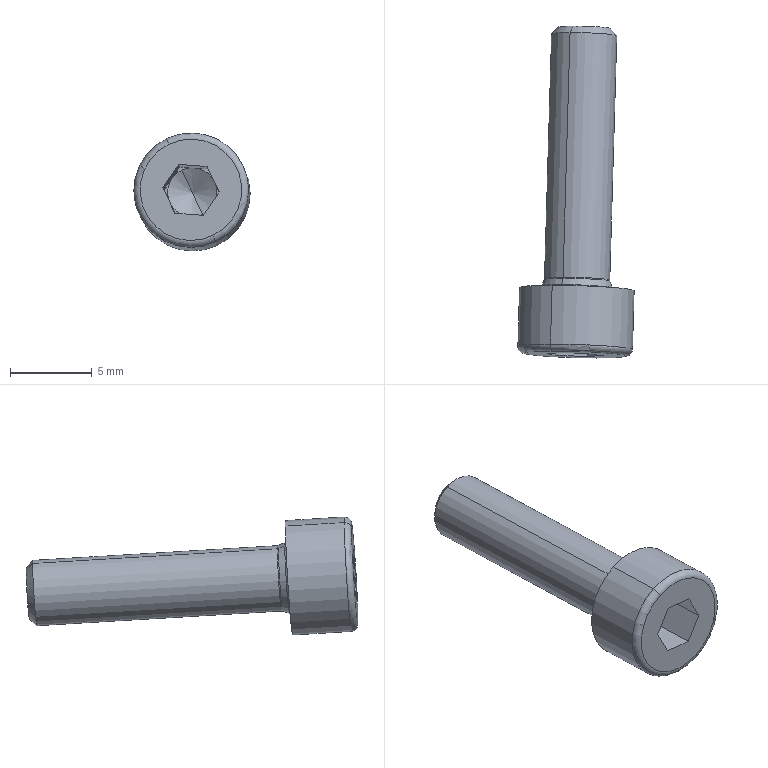Component | SolidWorks | HTCPA32_S5M100_12-1_Slotted_head_cap_screw_ISO_4762_M4x16-1 | 1 solid | 31 faces | box 7.1 x 20.27 x 7.2 mm | volume 332 mm3 | plane 15 | cone 6 | torus 6 | cylinder 4 | commonest cylinder face diameters 4 x2 7 x2
STEP:
#1=COLOUR_RGB('',0.7922,0.8196,0.9333);
#2=FILL_AREA_STYLE_COLOUR('',#1);
#3=FILL_AREA_STYLE('',(#2));
#4=SURFACE_STYLE_FILL_AREA(#3);
#5=SURFACE_SIDE_STYLE('',(#4));
#6=SURFACE_STYLE_USAGE(.BOTH.,#5);
#7=PRESENTATION_STYLE_ASSIGNMENT((#6));
#8=CARTESIAN_POINT('',(-1.2,11.445,21.934));
#9=VERTEX_POINT('',#8);
#10=CARTESIAN_POINT('',(-1.226,11.415,21.989));
#11=VERTEX_POINT('',#10);
#12=CARTESIAN_POINT('',(-1.226,11.415,21.989));
#13=DIRECTION('',(-0.3875,-0.4412,0.8094));
#14=VECTOR('',#13,39.37);
#15=LINE('',#12,#14);
#16=EDGE_CURVE('',#9,#11,#15,.T.);
#17=ORIENTED_EDGE('',*,*,#16,.F.);
#18=CARTESIAN_POINT('',(-1.175,11.407,21.883));
#19=VERTEX_POINT('',#18);
#20=CARTESIAN_POINT('',(-1.175,11.407,21.883));
#21=DIRECTION('',(0.3587,-0.5566,-0.7494));
#22=VECTOR('',#21,39.37);
#23=LINE('',#20,#22);
#24=EDGE_CURVE('',#9,#19,#23,.T.);
#25=ORIENTED_EDGE('',*,*,#24,.T.);
#26=CARTESIAN_POINT('',(-1.152,11.408,21.903));
#27=VERTEX_POINT('',#26);
#28=CARTESIAN_POINT('',(-1.201,11.411,21.936));
#29=DIRECTION('',(-0.02875,-0.9978,0.06006));
#30=DIRECTION('',(-0.4308,0.06659,0.9));
#31=AXIS2_PLACEMENT_3D('',#28,#29,#30);
#32=CIRCLE('',#31,0.05906);
#33=EDGE_CURVE('',#19,#27,#32,.T.);
#34=ORIENTED_EDGE('',*,*,#33,.T.);
#35=CARTESIAN_POINT('',(-1.147,11.411,21.962));
#36=VERTEX_POINT('',#35);
#37=CARTESIAN_POINT('',(-1.201,11.411,21.936));
#38=DIRECTION('',(-0.02875,-0.9978,0.06006));
#39=DIRECTION('',(-0.4308,0.06659,0.9));
#40=AXIS2_PLACEMENT_3D('',#37,#38,#39);
#41=CIRCLE('',#40,0.05906);
#42=EDGE_CURVE('',#27,#36,#41,.T.);
#43=ORIENTED_EDGE('',*,*,#42,.T.);
#44=CARTESIAN_POINT('',(-1.196,11.415,21.995));
#45=VERTEX_POINT('',#44);
#46=CARTESIAN_POINT('',(-1.201,11.411,21.936));
#47=DIRECTION('',(-0.02875,-0.9978,0.06006));
#48=DIRECTION('',(-0.4308,0.06659,0.9));
#49=AXIS2_PLACEMENT_3D('',#46,#47,#48);
#50=CIRCLE('',#49,0.05906);
#51=EDGE_CURVE('',#36,#45,#50,.T.);
#52=ORIENTED_EDGE('',*,*,#51,.T.);
#53=CARTESIAN_POINT('',(-1.201,11.411,21.936));
#54=DIRECTION('',(-0.02875,-0.9978,0.06006));
#55=DIRECTION('',(-0.4308,0.06659,0.9));
#56=AXIS2_PLACEMENT_3D('',#53,#54,#55);
#57=CIRCLE('',#56,0.05906);
#58=EDGE_CURVE('',#45,#11,#57,.T.);
#59=ORIENTED_EDGE('',*,*,#58,.T.);
#60=EDGE_LOOP('',(#17,#25,#34,#43,#52,#59));
#61=FACE_OUTER_BOUND('',#60,.T.);
#62=CARTESIAN_POINT('',(-1.201,11.411,21.936));
#63=DIRECTION('',(-0.02875,-0.9978,0.06006));
#64=DIRECTION('',(-0.4308,0.06659,0.9));
#65=AXIS2_PLACEMENT_3D('',#62,#63,#64);
#66=CONICAL_SURFACE('',#65,0.05906,1.047);
#67=ADVANCED_FACE('',(#61),#66,.F.);
#68=CARTESIAN_POINT('',(-1.208,12.099,21.951));
#69=VERTEX_POINT('',#68);
#70=CARTESIAN_POINT('',(-1.154,12.091,21.839));
#71=VERTEX_POINT('',#70);
#72=CARTESIAN_POINT('',(-1.181,12.095,21.895));
#73=DIRECTION('',(-0.02875,-0.9978,0.06006));
#74=DIRECTION('',(-0.4308,0.06659,0.9));
#75=AXIS2_PLACEMENT_3D('',#72,#73,#74);
#76=CIRCLE('',#75,0.06183);
#77=EDGE_CURVE('',#69,#71,#76,.T.);
#78=ORIENTED_EDGE('',*,*,#77,.T.);
#79=CARTESIAN_POINT('',(-1.147,12.073,21.825));
#80=VERTEX_POINT('',#79);
#81=CARTESIAN_POINT('',(-1.154,12.091,21.839));
#82=DIRECTION('',(0.2843,-0.7526,-0.5939));
#83=VECTOR('',#82,39.37);
#84=LINE('',#81,#83);
#85=EDGE_CURVE('',#71,#80,#84,.T.);
#86=ORIENTED_EDGE('',*,*,#85,.T.);
#87=CARTESIAN_POINT('',(-1.215,12.083,21.967));
#88=VERTEX_POINT('',#87);
#89=CARTESIAN_POINT('',(-1.181,12.078,21.896));
#90=DIRECTION('',(-0.02875,-0.9978,0.06006));
#91=DIRECTION('',(-0.4308,0.06659,0.9));
#92=AXIS2_PLACEMENT_3D('',#89,#90,#91);
#93=CIRCLE('',#92,0.07874);
#94=EDGE_CURVE('',#88,#80,#93,.T.);
#95=ORIENTED_EDGE('',*,*,#94,.F.);
#96=CARTESIAN_POINT('',(-1.208,12.099,21.951));
#97=DIRECTION('',(-0.325,-0.6585,0.6788));
#98=VECTOR('',#97,39.37);
#99=LINE('',#96,#98);
#100=EDGE_CURVE('',#69,#88,#99,.T.);
#101=ORIENTED_EDGE('',*,*,#100,.F.);
#102=EDGE_LOOP('',(#78,#86,#95,#101));
#103=FACE_OUTER_BOUND('',#102,.T.);
#104=CARTESIAN_POINT('',(-1.181,12.095,21.895));
#105=DIRECTION('',(-0.02875,-0.9978,0.06006));
#106=DIRECTION('',(-0.4308,0.06659,0.9));
#107=AXIS2_PLACEMENT_3D('',#104,#105,#106);
#108=CONICAL_SURFACE('',#107,0.06183,0.7854);
#109=ADVANCED_FACE('',(#103),#108,.T.);
#110=ORIENTED_EDGE('',*,*,#94,.T.);
#111=CARTESIAN_POINT('',(-1.164,11.485,21.861));
#112=VERTEX_POINT('',#111);
#113=CARTESIAN_POINT('',(-1.147,12.09,21.824));
#114=DIRECTION('',(-0.02875,-0.9978,0.06006));
#115=VECTOR('',#114,39.37);
#116=LINE('',#113,#115);
#117=EDGE_CURVE('',#80,#112,#116,.T.);
#118=ORIENTED_EDGE('',*,*,#117,.T.);
#119=CARTESIAN_POINT('',(-1.232,11.495,22.002));
#120=VERTEX_POINT('',#119);
#121=CARTESIAN_POINT('',(-1.198,11.49,21.931));
#122=DIRECTION('',(-0.02875,-0.9978,0.06006));
#123=DIRECTION('',(-0.4308,0.06659,0.9));
#124=AXIS2_PLACEMENT_3D('',#121,#122,#123);
#125=CIRCLE('',#124,0.07874);
#126=EDGE_CURVE('',#120,#112,#125,.T.);
#127=ORIENTED_EDGE('',*,*,#126,.F.);
#128=CARTESIAN_POINT('',(-1.215,12.1,21.966));
#129=DIRECTION('',(-0.02875,-0.9978,0.06006));
#130=VECTOR('',#129,39.37);
#131=LINE('',#128,#130);
#132=EDGE_CURVE('',#88,#120,#131,.T.);
#133=ORIENTED_EDGE('',*,*,#132,.F.);
#134=EDGE_LOOP('',(#110,#118,#127,#133));
#135=FACE_OUTER_BOUND('',#134,.T.);
#136=CARTESIAN_POINT('',(-1.181,12.095,21.895));
#137=DIRECTION('',(-0.02875,-0.9978,0.06006));
#138=DIRECTION('',(-0.4308,0.06659,0.9));
#139=AXIS2_PLACEMENT_3D('',#136,#137,#138);
#140=CYLINDRICAL_SURFACE('',#139,0.07874);
#141=ADVANCED_FACE('',(#135),#140,.T.);
#142=CARTESIAN_POINT('',(-1.164,11.482,21.86));
#143=VERTEX_POINT('',#142);
#144=CARTESIAN_POINT('',(-1.233,11.492,22.003));
#145=VERTEX_POINT('',#144);
#146=CARTESIAN_POINT('',(-1.198,11.487,21.932));
#147=DIRECTION('',(-0.02875,-0.9978,0.06006));
#148=DIRECTION('',(-0.4308,0.06659,0.9));
#149=AXIS2_PLACEMENT_3D('',#146,#147,#148);
#150=CIRCLE('',#149,0.07924);
#151=EDGE_CURVE('',#143,#145,#150,.T.);
#152=ORIENTED_EDGE('',*,*,#151,.F.);
#153=CARTESIAN_POINT('',(-1.161,11.484,21.853));
#154=DIRECTION('',(-0.902,0.,-0.4318));
#155=DIRECTION('',(-0.4318,0.,0.902));
#156=AXIS2_PLACEMENT_3D('',#153,#154,#155);
#157=CIRCLE('',#156,0.007874);
#158=EDGE_CURVE('',#143,#112,#157,.T.);
#159=ORIENTED_EDGE('',*,*,#158,.T.);
#160=CARTESIAN_POINT('',(-1.198,11.49,21.931));
#161=DIRECTION('',(-0.02875,-0.9978,0.06006));
#162=DIRECTION('',(-0.4308,0.06659,0.9));
#163=AXIS2_PLACEMENT_3D('',#160,#161,#162);
#164=CIRCLE('',#163,0.07874);
#165=EDGE_CURVE('',#112,#120,#164,.T.);
#166=ORIENTED_EDGE('',*,*,#165,.T.);
#167=CARTESIAN_POINT('',(-1.236,11.496,22.009));
#168=DIRECTION('',(0.902,-0.,0.4318));
#169=DIRECTION('',(0.4318,0.,-0.902));
#170=AXIS2_PLACEMENT_3D('',#167,#168,#169);
#171=CIRCLE('',#170,0.007874);
#172=EDGE_CURVE('',#145,#120,#171,.T.);
#173=ORIENTED_EDGE('',*,*,#172,.F.);
#174=EDGE_LOOP('',(#152,#159,#166,#173));
#175=FACE_OUTER_BOUND('',#174,.T.);
#176=CARTESIAN_POINT('',(-1.198,11.49,21.931));
#177=DIRECTION('',(-0.02875,-0.9978,0.06006));
#178=DIRECTION('',(-0.4308,0.06659,0.9));
#179=AXIS2_PLACEMENT_3D('',#176,#177,#178);
#180=TOROIDAL_SURFACE('',#179,0.08661,0.007874);
#181=ADVANCED_FACE('',(#175),#180,.F.);
#182=CARTESIAN_POINT('',(-1.198,11.487,21.932));
#183=DIRECTION('',(-0.02875,-0.9978,0.06006));
#184=DIRECTION('',(-0.4308,0.06659,0.9));
#185=AXIS2_PLACEMENT_3D('',#182,#183,#184);
#186=CIRCLE('',#185,0.07924);
#187=EDGE_CURVE('',#145,#143,#186,.T.);
#188=ORIENTED_EDGE('',*,*,#187,.T.);
#189=CARTESIAN_POINT('',(-1.162,11.466,21.856));
#190=VERTEX_POINT('',#189);
#191=CARTESIAN_POINT('',(-1.164,11.482,21.86));
#192=DIRECTION('',(0.1244,-0.9576,-0.2598));
#193=VECTOR('',#192,39.37);
#194=LINE('',#191,#193);
#195=EDGE_CURVE('',#143,#190,#194,.T.);
#196=ORIENTED_EDGE('',*,*,#195,.T.);
#197=CARTESIAN_POINT('',(-1.236,11.477,22.009));
#198=VERTEX_POINT('',#197);
#199=CARTESIAN_POINT('',(-1.199,11.471,21.933));
#200=DIRECTION('',(-0.02875,-0.9978,0.06006));
#201=DIRECTION('',(-0.4308,0.06659,0.9));
#202=AXIS2_PLACEMENT_3D('',#199,#200,#201);
#203=CIRCLE('',#202,0.08515);
#204=EDGE_CURVE('',#198,#190,#203,.T.);
#205=ORIENTED_EDGE('',*,*,#204,.F.);
#206=CARTESIAN_POINT('',(-1.233,11.492,22.003));
#207=DIRECTION('',(-0.1782,-0.9109,0.3722));
#208=VECTOR('',#207,39.37);
#209=LINE('',#206,#208);
#210=EDGE_CURVE('',#145,#198,#209,.T.);
#211=ORIENTED_EDGE('',*,*,#210,.F.);
#212=EDGE_LOOP('',(#188,#196,#205,#211));
#213=FACE_OUTER_BOUND('',#212,.T.);
#214=CARTESIAN_POINT('',(-1.198,11.487,21.932));
#215=DIRECTION('',(-0.02875,-0.9978,0.06006));
#216=DIRECTION('',(-0.4308,0.06659,0.9));
#217=AXIS2_PLACEMENT_3D('',#214,#215,#216);
#218=CONICAL_SURFACE('',#217,0.07924,0.3588);
#219=ADVANCED_FACE('',(#213),#218,.T.);
#220=CARTESIAN_POINT('',(-1.159,11.46,21.85));
#221=VERTEX_POINT('',#220);
#222=CARTESIAN_POINT('',(-1.239,11.472,22.016));
#223=VERTEX_POINT('',#222);
#224=CARTESIAN_POINT('',(-1.199,11.466,21.933));
#225=DIRECTION('',(-0.02875,-0.9978,0.06006));
#226=DIRECTION('',(-0.4308,0.06659,0.9));
#227=AXIS2_PLACEMENT_3D('',#224,#225,#226);
#228=CIRCLE('',#227,0.09252);
#229=EDGE_CURVE('',#221,#223,#228,.T.);
#230=ORIENTED_EDGE('',*,*,#229,.F.);
#231=CARTESIAN_POINT('',(-1.159,11.468,21.849));
#232=DIRECTION('',(-0.902,0.,-0.4318));
#233=DIRECTION('',(-0.4318,0.,0.902));
#234=AXIS2_PLACEMENT_3D('',#231,#232,#233);
#235=CIRCLE('',#234,0.007874);
#236=EDGE_CURVE('',#221,#190,#235,.T.);
#237=ORIENTED_EDGE('',*,*,#236,.T.);
#238=CARTESIAN_POINT('',(-1.199,11.471,21.933));
#239=DIRECTION('',(-0.02875,-0.9978,0.06006));
#240=DIRECTION('',(-0.4308,0.06659,0.9));
#241=AXIS2_PLACEMENT_3D('',#238,#239,#240);
#242=CIRCLE('',#241,0.08515);
#243=EDGE_CURVE('',#190,#198,#242,.T.);
#244=ORIENTED_EDGE('',*,*,#243,.T.);
#245=CARTESIAN_POINT('',(-1.239,11.48,22.016));
#246=DIRECTION('',(0.902,-0.,0.4318));
#247=DIRECTION('',(0.4318,0.,-0.902));
#248=AXIS2_PLACEMENT_3D('',#245,#246,#247);
#249=CIRCLE('',#248,0.007874);
#250=EDGE_CURVE('',#223,#198,#249,.T.);
#251=ORIENTED_EDGE('',*,*,#250,.F.);
#252=EDGE_LOOP('',(#230,#237,#244,#251));
#253=FACE_OUTER_BOUND('',#252,.T.);
#254=CARTESIAN_POINT('',(-1.199,11.474,21.932));
#255=DIRECTION('',(-0.02875,-0.9978,0.06006));
#256=DIRECTION('',(-0.4308,0.06659,0.9));
#257=AXIS2_PLACEMENT_3D('',#254,#255,#256);
#258=TOROIDAL_SURFACE('',#257,0.09252,0.007874);
#259=ADVANCED_FACE('',(#253),#258,.F.);
#260=CARTESIAN_POINT('',(-1.258,11.475,22.057));
#261=VERTEX_POINT('',#260);
#262=CARTESIAN_POINT('',(-1.14,11.457,21.809));
#263=VERTEX_POINT('',#262);
#264=CARTESIAN_POINT('',(-1.199,11.466,21.933));
#265=DIRECTION('',(-0.02875,-0.9978,0.06006));
#266=DIRECTION('',(-0.4308,0.06659,0.9));
#267=AXIS2_PLACEMENT_3D('',#264,#265,#266);
#268=CIRCLE('',#267,0.1378);
#269=EDGE_CURVE('',#261,#263,#268,.T.);
#270=ORIENTED_EDGE('',*,*,#269,.T.);
#271=CARTESIAN_POINT('',(-1.144,11.316,21.817));
#272=VERTEX_POINT('',#271);
#273=CARTESIAN_POINT('',(-1.122,12.086,21.771));
#274=DIRECTION('',(-0.02875,-0.9978,0.06006));
#275=VECTOR('',#274,39.37);
#276=LINE('',#273,#275);
#277=EDGE_CURVE('',#263,#272,#276,.T.);
#278=ORIENTED_EDGE('',*,*,#277,.T.);
#279=CARTESIAN_POINT('',(-1.262,11.334,22.065));
#280=VERTEX_POINT('',#279);
#281=CARTESIAN_POINT('',(-1.203,11.325,21.941));
#282=DIRECTION('',(-0.02875,-0.9978,0.06006));
#283=DIRECTION('',(-0.4308,0.06659,0.9));
#284=AXIS2_PLACEMENT_3D('',#281,#282,#283);
#285=CIRCLE('',#284,0.1378);
#286=EDGE_CURVE('',#280,#272,#285,.T.);
#287=ORIENTED_EDGE('',*,*,#286,.F.);
#288=CARTESIAN_POINT('',(-1.24,12.104,22.019));
#289=DIRECTION('',(-0.02875,-0.9978,0.06006));
#290=VECTOR('',#289,39.37);
#291=LINE('',#288,#290);
#292=EDGE_CURVE('',#261,#280,#291,.T.);
#293=ORIENTED_EDGE('',*,*,#292,.F.);
#294=EDGE_LOOP('',(#270,#278,#287,#293));
#295=FACE_OUTER_BOUND('',#294,.T.);
#296=CARTESIAN_POINT('',(-1.181,12.095,21.895));
#297=DIRECTION('',(-0.02875,-0.9978,0.06006));
#298=DIRECTION('',(-0.4308,0.06659,0.9));
#299=AXIS2_PLACEMENT_3D('',#296,#297,#298);
#300=CYLINDRICAL_SURFACE('',#299,0.1378);
#301=ADVANCED_FACE('',(#295),#300,.T.);
#302=ORIENTED_EDGE('',*,*,#286,.T.);
#303=CARTESIAN_POINT('',(-1.151,11.301,21.832));
#304=VERTEX_POINT('',#303);
#305=CARTESIAN_POINT('',(-1.151,11.317,21.832));
#306=DIRECTION('',(-0.902,0.,-0.4318));
#307=DIRECTION('',(-0.4318,0.,0.902));
#308=AXIS2_PLACEMENT_3D('',#305,#306,#307);
#309=CIRCLE('',#308,0.01575);
#310=EDGE_CURVE('',#272,#304,#309,.T.);
#311=ORIENTED_EDGE('',*,*,#310,.T.);
#312=CARTESIAN_POINT('',(-1.256,11.317,22.052));
#313=VERTEX_POINT('',#312);
#314=CARTESIAN_POINT('',(-1.204,11.309,21.942));
#315=DIRECTION('',(-0.02875,-0.9978,0.06006));
#316=DIRECTION('',(-0.4308,0.06659,0.9));
#317=AXIS2_PLACEMENT_3D('',#314,#315,#316);
#318=CIRCLE('',#317,0.122);
#319=EDGE_CURVE('',#313,#304,#318,.T.);
#320=ORIENTED_EDGE('',*,*,#319,.F.);
#321=CARTESIAN_POINT('',(-1.256,11.333,22.051));
#322=DIRECTION('',(0.902,-0.,0.4318));
#323=DIRECTION('',(0.4318,0.,-0.902));
#324=AXIS2_PLACEMENT_3D('',#321,#322,#323);
#325=CIRCLE('',#324,0.01575);
#326=EDGE_CURVE('',#280,#313,#325,.T.);
#327=ORIENTED_EDGE('',*,*,#326,.F.);
#328=EDGE_LOOP('',(#302,#311,#320,#327));
#329=FACE_OUTER_BOUND('',#328,.T.);
#330=CARTESIAN_POINT('',(-1.203,11.325,21.941));
#331=DIRECTION('',(-0.02875,-0.9978,0.06006));
#332=DIRECTION('',(-0.4308,0.06659,0.9));
#333=AXIS2_PLACEMENT_3D('',#330,#331,#332);
#334=TOROIDAL_SURFACE('',#333,0.122,0.01575);
#335=ADVANCED_FACE('',(#329),#334,.T.);
#336=CARTESIAN_POINT('',(-1.233,11.314,22.004));
#337=VERTEX_POINT('',#336);
#338=CARTESIAN_POINT('',(-1.165,11.311,21.998));
#339=VERTEX_POINT('',#338);
#340=CARTESIAN_POINT('',(-1.17,11.312,21.999));
#341=DIRECTION('',(0.9965,-0.03329,-0.07605));
#342=VECTOR('',#341,39.37);
#343=LINE('',#340,#342);
#344=EDGE_CURVE('',#337,#339,#343,.T.);
#345=ORIENTED_EDGE('',*,*,#344,.T.);
#346=CARTESIAN_POINT('',(-1.136,11.307,21.937));
#347=VERTEX_POINT('',#346);
#348=CARTESIAN_POINT('',(-1.125,11.305,21.915));
#349=DIRECTION('',(0.4308,-0.06659,-0.9));
#350=VECTOR('',#349,39.37);
#351=LINE('',#348,#350);
#352=EDGE_CURVE('',#339,#347,#351,.T.);
#353=ORIENTED_EDGE('',*,*,#352,.T.);
#354=CARTESIAN_POINT('',(-1.174,11.305,21.881));
#355=VERTEX_POINT('',#354);
#356=CARTESIAN_POINT('',(-1.172,11.305,21.885));
#357=DIRECTION('',(-0.5657,-0.03329,-0.8239));
#358=VECTOR('',#357,39.37);
#359=LINE('',#356,#358);
#360=EDGE_CURVE('',#347,#355,#359,.T.);
#361=ORIENTED_EDGE('',*,*,#360,.T.);
#362=CARTESIAN_POINT('',(-1.242,11.307,21.886));
#363=VERTEX_POINT('',#362);
#364=CARTESIAN_POINT('',(-1.179,11.305,21.881));
#365=DIRECTION('',(-0.9965,0.03329,0.07605));
#366=VECTOR('',#365,39.37);
#367=LINE('',#364,#366);
#368=EDGE_CURVE('',#355,#363,#367,.T.);
#369=ORIENTED_EDGE('',*,*,#368,.T.);
#370=CARTESIAN_POINT('',(-1.271,11.311,21.947));
#371=VERTEX_POINT('',#370);
#372=CARTESIAN_POINT('',(-1.231,11.305,21.864));
#373=DIRECTION('',(-0.4308,0.06659,0.9));
#374=VECTOR('',#373,39.37);
#375=LINE('',#372,#374);
#376=EDGE_CURVE('',#363,#371,#375,.T.);
#377=ORIENTED_EDGE('',*,*,#376,.T.);
#378=CARTESIAN_POINT('',(-1.269,11.312,21.951));
#379=DIRECTION('',(0.5657,0.03329,0.8239));
#380=VECTOR('',#379,39.37);
#381=LINE('',#378,#380);
#382=EDGE_CURVE('',#371,#337,#381,.T.);
#383=ORIENTED_EDGE('',*,*,#382,.T.);
#384=EDGE_LOOP('',(#345,#353,#361,#369,#377,#383));
#385=FACE_BOUND('',#384,.T.);
#386=ORIENTED_EDGE('',*,*,#319,.T.);
#387=CARTESIAN_POINT('',(-1.204,11.309,21.942));
#388=DIRECTION('',(-0.02875,-0.9978,0.06006));
#389=DIRECTION('',(-0.4308,0.06659,0.9));
#390=AXIS2_PLACEMENT_3D('',#387,#388,#389);
#391=CIRCLE('',#390,0.122);
#392=EDGE_CURVE('',#304,#313,#391,.T.);
#393=ORIENTED_EDGE('',*,*,#392,.T.);
#394=EDGE_LOOP('',(#386,#393));
#395=FACE_OUTER_BOUND('',#394,.T.);
#396=CARTESIAN_POINT('',(-1.178,11.305,21.889));
#397=DIRECTION('',(0.02875,0.9978,-0.06006));
#398=DIRECTION('',(0.4308,-0.06659,-0.9));
#399=AXIS2_PLACEMENT_3D('',#396,#397,#398);
#400=PLANE('',#399);
#401=ADVANCED_FACE('',(#385,#395),#400,.F.);
#402=ORIENTED_EDGE('',*,*,#310,.F.);
#403=CARTESIAN_POINT('',(-1.203,11.325,21.941));
#404=DIRECTION('',(-0.02875,-0.9978,0.06006));
#405=DIRECTION('',(-0.4308,0.06659,0.9));
#406=AXIS2_PLACEMENT_3D('',#403,#404,#405);
#407=CIRCLE('',#406,0.1378);
#408=EDGE_CURVE('',#272,#280,#407,.T.);
#409=ORIENTED_EDGE('',*,*,#408,.T.);
#410=ORIENTED_EDGE('',*,*,#326,.T.);
#411=ORIENTED_EDGE('',*,*,#392,.F.);
#412=EDGE_LOOP('',(#402,#409,#410,#411));
#413=FACE_OUTER_BOUND('',#412,.T.);
#414=CARTESIAN_POINT('',(-1.203,11.325,21.941));
#415=DIRECTION('',(-0.02875,-0.9978,0.06006));
#416=DIRECTION('',(-0.4308,0.06659,0.9));
#417=AXIS2_PLACEMENT_3D('',#414,#415,#416);
#418=TOROIDAL_SURFACE('',#417,0.122,0.01575);
#419=ADVANCED_FACE('',(#413),#418,.T.);
#420=ORIENTED_EDGE('',*,*,#277,.F.);
#421=CARTESIAN_POINT('',(-1.199,11.466,21.933));
#422=DIRECTION('',(-0.02875,-0.9978,0.06006));
#423=DIRECTION('',(-0.4308,0.06659,0.9));
#424=AXIS2_PLACEMENT_3D('',#421,#422,#423);
#425=CIRCLE('',#424,0.1378);
#426=EDGE_CURVE('',#263,#261,#425,.T.);
#427=ORIENTED_EDGE('',*,*,#426,.T.);
#428=ORIENTED_EDGE('',*,*,#292,.T.);
#429=ORIENTED_EDGE('',*,*,#408,.F.);
#430=EDGE_LOOP('',(#420,#427,#428,#429));
#431=FACE_OUTER_BOUND('',#430,.T.);
#432=CARTESIAN_POINT('',(-1.181,12.095,21.895));
#433=DIRECTION('',(-0.02875,-0.9978,0.06006));
#434=DIRECTION('',(-0.4308,0.06659,0.9));
#435=AXIS2_PLACEMENT_3D('',#432,#433,#434);
#436=CYLINDRICAL_SURFACE('',#435,0.1378);
#437=ADVANCED_FACE('',(#431),#436,.T.);
#438=ORIENTED_EDGE('',*,*,#269,.F.);
#439=ORIENTED_EDGE('',*,*,#426,.F.);
#440=EDGE_LOOP('',(#438,#439));
#441=FACE_OUTER_BOUND('',#440,.T.);
#442=CARTESIAN_POINT('',(-1.199,11.466,21.933));
#443=DIRECTION('',(-0.02875,-0.9978,0.06006));
#444=DIRECTION('',(-0.4308,0.06659,0.9));
#445=AXIS2_PLACEMENT_3D('',#442,#443,#444);
#446=CIRCLE('',#445,0.09252);
#447=EDGE_CURVE('',#223,#221,#446,.T.);
#448=ORIENTED_EDGE('',*,*,#447,.T.);
#449=ORIENTED_EDGE('',*,*,#229,.T.);
#450=EDGE_LOOP('',(#448,#449));
#451=FACE_BOUND('',#450,.T.);
#452=CARTESIAN_POINT('',(-1.14,11.457,21.809));
#453=DIRECTION('',(-0.02875,-0.9978,0.06006));
#454=DIRECTION('',(-0.4308,0.06659,0.9));
#455=AXIS2_PLACEMENT_3D('',#452,#453,#454);
#456=PLANE('',#455);
#457=ADVANCED_FACE('',(#441,#451),#456,.F.);
#458=ORIENTED_EDGE('',*,*,#236,.F.);
#459=ORIENTED_EDGE('',*,*,#447,.F.);
#460=ORIENTED_EDGE('',*,*,#250,.T.);
#461=ORIENTED_EDGE('',*,*,#204,.T.);
#462=EDGE_LOOP('',(#458,#459,#460,#461));
#463=FACE_OUTER_BOUND('',#462,.T.);
#464=CARTESIAN_POINT('',(-1.199,11.474,21.932));
#465=DIRECTION('',(-0.02875,-0.9978,0.06006));
#466=DIRECTION('',(-0.4308,0.06659,0.9));
#467=AXIS2_PLACEMENT_3D('',#464,#465,#466);
#468=TOROIDAL_SURFACE('',#467,0.09252,0.007874);
#469=ADVANCED_FACE('',(#463),#468,.F.);
#470=ORIENTED_EDGE('',*,*,#195,.F.);
#471=ORIENTED_EDGE('',*,*,#151,.T.);
#472=ORIENTED_EDGE('',*,*,#210,.T.);
#473=ORIENTED_EDGE('',*,*,#243,.F.);
#474=EDGE_LOOP('',(#470,#471,#472,#473));
#475=FACE_OUTER_BOUND('',#474,.T.);
#476=CARTESIAN_POINT('',(-1.198,11.487,21.932));
#477=DIRECTION('',(-0.02875,-0.9978,0.06006));
#478=DIRECTION('',(-0.4308,0.06659,0.9));
#479=AXIS2_PLACEMENT_3D('',#476,#477,#478);
#480=CONICAL_SURFACE('',#479,0.07924,0.3588);
#481=ADVANCED_FACE('',(#475),#480,.T.);
#482=ORIENTED_EDGE('',*,*,#158,.F.);
#483=ORIENTED_EDGE('',*,*,#187,.F.);
#484=ORIENTED_EDGE('',*,*,#172,.T.);
#485=ORIENTED_EDGE('',*,*,#126,.T.);
#486=EDGE_LOOP('',(#482,#483,#484,#485));
#487=FACE_OUTER_BOUND('',#486,.T.);
#488=CARTESIAN_POINT('',(-1.198,11.49,21.931));
#489=DIRECTION('',(-0.02875,-0.9978,0.06006));
#490=DIRECTION('',(-0.4308,0.06659,0.9));
#491=AXIS2_PLACEMENT_3D('',#488,#489,#490);
#492=TOROIDAL_SURFACE('',#491,0.08661,0.007874);
#493=ADVANCED_FACE('',(#487),#492,.F.);
#494=ORIENTED_EDGE('',*,*,#117,.F.);
#495=CARTESIAN_POINT('',(-1.181,12.078,21.896));
#496=DIRECTION('',(-0.02875,-0.9978,0.06006));
#497=DIRECTION('',(-0.4308,0.06659,0.9));
#498=AXIS2_PLACEMENT_3D('',#495,#496,#497);
#499=CIRCLE('',#498,0.07874);
#500=EDGE_CURVE('',#80,#88,#499,.T.);
#501=ORIENTED_EDGE('',*,*,#500,.T.);
#502=ORIENTED_EDGE('',*,*,#132,.T.);
#503=ORIENTED_EDGE('',*,*,#165,.F.);
#504=EDGE_LOOP('',(#494,#501,#502,#503));
#505=FACE_OUTER_BOUND('',#504,.T.);
#506=CARTESIAN_POINT('',(-1.181,12.095,21.895));
#507=DIRECTION('',(-0.02875,-0.9978,0.06006));
#508=DIRECTION('',(-0.4308,0.06659,0.9));
#509=AXIS2_PLACEMENT_3D('',#506,#507,#508);
#510=CYLINDRICAL_SURFACE('',#509,0.07874);
#511=ADVANCED_FACE('',(#505),#510,.T.);
#512=ORIENTED_EDGE('',*,*,#85,.F.);
#513=CARTESIAN_POINT('',(-1.181,12.095,21.895));
#514=DIRECTION('',(-0.02875,-0.9978,0.06006));
#515=DIRECTION('',(-0.4308,0.06659,0.9));
#516=AXIS2_PLACEMENT_3D('',#513,#514,#515);
#517=CIRCLE('',#516,0.06183);
#518=EDGE_CURVE('',#71,#69,#517,.T.);
#519=ORIENTED_EDGE('',*,*,#518,.T.);
#520=ORIENTED_EDGE('',*,*,#100,.T.);
#521=ORIENTED_EDGE('',*,*,#500,.F.);
#522=EDGE_LOOP('',(#512,#519,#520,#521));
#523=FACE_OUTER_BOUND('',#522,.T.);
#524=CARTESIAN_POINT('',(-1.181,12.095,21.895));
#525=DIRECTION('',(-0.02875,-0.9978,0.06006));
#526=DIRECTION('',(-0.4308,0.06659,0.9));
#527=AXIS2_PLACEMENT_3D('',#524,#525,#526);
#528=CONICAL_SURFACE('',#527,0.06183,0.7854);
#529=ADVANCED_FACE('',(#523),#528,.T.);
#530=ORIENTED_EDGE('',*,*,#77,.F.);
#531=ORIENTED_EDGE('',*,*,#518,.F.);
#532=EDGE_LOOP('',(#530,#531));
#533=FACE_OUTER_BOUND('',#532,.T.);
#534=CARTESIAN_POINT('',(-1.154,12.091,21.839));
#535=DIRECTION('',(-0.02875,-0.9978,0.06006));
#536=DIRECTION('',(-0.4308,0.06659,0.9));
#537=AXIS2_PLACEMENT_3D('',#534,#535,#536);
#538=PLANE('',#537);
#539=ADVANCED_FACE('',(#533),#538,.F.);
#540=CARTESIAN_POINT('',(-1.162,11.414,21.992));
#541=VERTEX_POINT('',#540);
#542=CARTESIAN_POINT('',(-1.162,11.414,21.992));
#543=DIRECTION('',(0.4308,-0.06659,-0.9));
#544=VECTOR('',#543,39.37);
#545=LINE('',#542,#544);
#546=EDGE_CURVE('',#541,#36,#545,.T.);
#547=ORIENTED_EDGE('',*,*,#546,.F.);
#548=CARTESIAN_POINT('',(-1.23,11.416,21.998));
#549=DIRECTION('',(0.9965,-0.03329,-0.07605));
#550=VECTOR('',#549,39.37);
#551=LINE('',#548,#550);
#552=EDGE_CURVE('',#45,#541,#551,.T.);
#553=ORIENTED_EDGE('',*,*,#552,.F.);
#554=ORIENTED_EDGE('',*,*,#51,.F.);
#555=EDGE_LOOP('',(#547,#553,#554));
#556=FACE_OUTER_BOUND('',#555,.T.);
#557=CARTESIAN_POINT('',(-1.201,11.411,21.936));
#558=DIRECTION('',(0.02875,0.9978,-0.06006));
#559=DIRECTION('',(0.902,-0.,0.4318));
#560=AXIS2_PLACEMENT_3D('',#557,#558,#559);
#561=PLANE('',#560);
#562=ADVANCED_FACE('',(#556),#561,.F.);
#563=CARTESIAN_POINT('',(-1.23,11.416,21.998));
#564=VERTEX_POINT('',#563);
#565=CARTESIAN_POINT('',(-1.23,11.416,21.998));
#566=DIRECTION('',(0.9965,-0.03329,-0.07605));
#567=VECTOR('',#566,39.37);
#568=LINE('',#565,#567);
#569=EDGE_CURVE('',#564,#45,#568,.T.);
#570=ORIENTED_EDGE('',*,*,#569,.F.);
#571=CARTESIAN_POINT('',(-1.249,11.415,21.969));
#572=VERTEX_POINT('',#571);
#573=CARTESIAN_POINT('',(-1.269,11.414,21.941));
#574=DIRECTION('',(0.5657,0.03329,0.8239));
#575=VECTOR('',#574,39.37);
#576=LINE('',#573,#575);
#577=EDGE_CURVE('',#572,#564,#576,.T.);
#578=ORIENTED_EDGE('',*,*,#577,.F.);
#579=CARTESIAN_POINT('',(-1.201,11.411,21.936));
#580=DIRECTION('',(-0.02875,-0.9978,0.06006));
#581=DIRECTION('',(-0.4308,0.06659,0.9));
#582=AXIS2_PLACEMENT_3D('',#579,#580,#581);
#583=CIRCLE('',#582,0.05906);
#584=EDGE_CURVE('',#11,#572,#583,.T.);
#585=ORIENTED_EDGE('',*,*,#584,.F.);
#586=ORIENTED_EDGE('',*,*,#58,.F.);
#587=EDGE_LOOP('',(#570,#578,#585,#586));
#588=FACE_OUTER_BOUND('',#587,.T.);
#589=CARTESIAN_POINT('',(-1.201,11.411,21.936));
#590=DIRECTION('',(0.02875,0.9978,-0.06006));
#591=DIRECTION('',(0.902,-0.,0.4318));
#592=AXIS2_PLACEMENT_3D('',#589,#590,#591);
#593=PLANE('',#592);
#594=ADVANCED_FACE('',(#588),#593,.F.);
#595=CARTESIAN_POINT('',(-1.269,11.414,21.941));
#596=VERTEX_POINT('',#595);
#597=CARTESIAN_POINT('',(-1.269,11.414,21.941));
#598=DIRECTION('',(0.5657,0.03329,0.8239));
#599=VECTOR('',#598,39.37);
#600=LINE('',#597,#599);
#601=EDGE_CURVE('',#596,#572,#600,.T.);
#602=ORIENTED_EDGE('',*,*,#601,.F.);
#603=CARTESIAN_POINT('',(-1.254,11.411,21.911));
#604=VERTEX_POINT('',#603);
#605=CARTESIAN_POINT('',(-1.239,11.409,21.88));
#606=DIRECTION('',(-0.4308,0.06659,0.9));
#607=VECTOR('',#606,39.37);
#608=LINE('',#605,#607);
#609=EDGE_CURVE('',#604,#596,#608,.T.);
#610=ORIENTED_EDGE('',*,*,#609,.F.);
#611=CARTESIAN_POINT('',(-1.201,11.411,21.936));
#612=DIRECTION('',(-0.02875,-0.9978,0.06006));
#613=DIRECTION('',(-0.4308,0.06659,0.9));
#614=AXIS2_PLACEMENT_3D('',#611,#612,#613);
#615=CIRCLE('',#614,0.05906);
#616=EDGE_CURVE('',#572,#604,#615,.T.);
#617=ORIENTED_EDGE('',*,*,#616,.F.);
#618=EDGE_LOOP('',(#602,#610,#617));
#619=FACE_OUTER_BOUND('',#618,.T.);
#620=CARTESIAN_POINT('',(-1.201,11.411,21.936));
#621=DIRECTION('',(0.02875,0.9978,-0.06006));
#622=DIRECTION('',(0.902,-0.,0.4318));
#623=AXIS2_PLACEMENT_3D('',#620,#621,#622);
#624=PLANE('',#623);
#625=ADVANCED_FACE('',(#619),#624,.F.);
#626=CARTESIAN_POINT('',(-1.239,11.409,21.88));
#627=VERTEX_POINT('',#626);
#628=CARTESIAN_POINT('',(-1.239,11.409,21.88));
#629=DIRECTION('',(-0.4308,0.06659,0.9));
#630=VECTOR('',#629,39.37);
#631=LINE('',#628,#630);
#632=EDGE_CURVE('',#627,#604,#631,.T.);
#633=ORIENTED_EDGE('',*,*,#632,.F.);
#634=CARTESIAN_POINT('',(-1.205,11.408,21.877));
#635=VERTEX_POINT('',#634);
#636=CARTESIAN_POINT('',(-1.171,11.407,21.875));
#637=DIRECTION('',(-0.9965,0.03329,0.07605));
#638=VECTOR('',#637,39.37);
#639=LINE('',#636,#638);
#640=EDGE_CURVE('',#635,#627,#639,.T.);
#641=ORIENTED_EDGE('',*,*,#640,.F.);
#642=CARTESIAN_POINT('',(-1.201,11.411,21.936));
#643=DIRECTION('',(-0.02875,-0.9978,0.06006));
#644=DIRECTION('',(-0.4308,0.06659,0.9));
#645=AXIS2_PLACEMENT_3D('',#642,#643,#644);
#646=CIRCLE('',#645,0.05906);
#647=EDGE_CURVE('',#604,#635,#646,.T.);
#648=ORIENTED_EDGE('',*,*,#647,.F.);
#649=EDGE_LOOP('',(#633,#641,#648));
#650=FACE_OUTER_BOUND('',#649,.T.);
#651=CARTESIAN_POINT('',(-1.201,11.411,21.936));
#652=DIRECTION('',(0.02875,0.9978,-0.06006));
#653=DIRECTION('',(0.902,-0.,0.4318));
#654=AXIS2_PLACEMENT_3D('',#651,#652,#653);
#655=PLANE('',#654);
#656=ADVANCED_FACE('',(#650),#655,.F.);
#657=CARTESIAN_POINT('',(-1.171,11.407,21.875));
#658=VERTEX_POINT('',#657);
#659=CARTESIAN_POINT('',(-1.171,11.407,21.875));
#660=DIRECTION('',(-0.9965,0.03329,0.07605));
#661=VECTOR('',#660,39.37);
#662=LINE('',#659,#661);
#663=EDGE_CURVE('',#658,#635,#662,.T.);
#664=ORIENTED_EDGE('',*,*,#663,.F.);
#665=CARTESIAN_POINT('',(-1.133,11.409,21.931));
#666=DIRECTION('',(-0.5657,-0.03329,-0.8239));
#667=VECTOR('',#666,39.37);
#668=LINE('',#665,#667);
#669=EDGE_CURVE('',#27,#658,#668,.T.);
#670=ORIENTED_EDGE('',*,*,#669,.F.);
#671=ORIENTED_EDGE('',*,*,#33,.F.);
#672=CARTESIAN_POINT('',(-1.201,11.411,21.936));
#673=DIRECTION('',(-0.02875,-0.9978,0.06006));
#674=DIRECTION('',(-0.4308,0.06659,0.9));
#675=AXIS2_PLACEMENT_3D('',#672,#673,#674);
#676=CIRCLE('',#675,0.05906);
#677=EDGE_CURVE('',#635,#19,#676,.T.);
#678=ORIENTED_EDGE('',*,*,#677,.F.);
#679=EDGE_LOOP('',(#664,#670,#671,#678));
#680=FACE_OUTER_BOUND('',#679,.T.);
#681=CARTESIAN_POINT('',(-1.201,11.411,21.936));
#682=DIRECTION('',(0.02875,0.9978,-0.06006));
#683=DIRECTION('',(0.902,-0.,0.4318));
#684=AXIS2_PLACEMENT_3D('',#681,#682,#683);
#685=PLANE('',#684);
#686=ADVANCED_FACE('',(#680),#685,.F.);
#687=CARTESIAN_POINT('',(-1.133,11.409,21.931));
#688=VERTEX_POINT('',#687);
#689=CARTESIAN_POINT('',(-1.133,11.409,21.931));
#690=DIRECTION('',(-0.5657,-0.03329,-0.8239));
#691=VECTOR('',#690,39.37);
#692=LINE('',#689,#691);
#693=EDGE_CURVE('',#688,#27,#692,.T.);
#694=ORIENTED_EDGE('',*,*,#693,.F.);
#695=CARTESIAN_POINT('',(-1.162,11.414,21.992));
#696=DIRECTION('',(0.4308,-0.06659,-0.9));
#697=VECTOR('',#696,39.37);
#698=LINE('',#695,#697);
#699=EDGE_CURVE('',#36,#688,#698,.T.);
#700=ORIENTED_EDGE('',*,*,#699,.F.);
#701=ORIENTED_EDGE('',*,*,#42,.F.);
#702=EDGE_LOOP('',(#694,#700,#701));
#703=FACE_OUTER_BOUND('',#702,.T.);
#704=CARTESIAN_POINT('',(-1.201,11.411,21.936));
#705=DIRECTION('',(0.02875,0.9978,-0.06006));
#706=DIRECTION('',(0.902,-0.,0.4318));
#707=AXIS2_PLACEMENT_3D('',#704,#705,#706);
#708=PLANE('',#707);
#709=ADVANCED_FACE('',(#703),#708,.F.);
#710=ORIENTED_EDGE('',*,*,#368,.F.);
#711=CARTESIAN_POINT('',(-1.176,11.25,21.884));
#712=DIRECTION('',(0.02875,0.9978,-0.06006));
#713=VECTOR('',#712,39.37);
#714=LINE('',#711,#713);
#715=EDGE_CURVE('',#355,#658,#714,.T.);
#716=ORIENTED_EDGE('',*,*,#715,.T.);
#717=ORIENTED_EDGE('',*,*,#663,.T.);
#718=ORIENTED_EDGE('',*,*,#640,.T.);
#719=CARTESIAN_POINT('',(-1.244,11.252,21.889));
#720=DIRECTION('',(0.02875,0.9978,-0.06006));
#721=VECTOR('',#720,39.37);
#722=LINE('',#719,#721);
#723=EDGE_CURVE('',#363,#627,#722,.T.);
#724=ORIENTED_EDGE('',*,*,#723,.F.);
#725=EDGE_LOOP('',(#710,#716,#717,#718,#724));
#726=FACE_OUTER_BOUND('',#725,.T.);
#727=CARTESIAN_POINT('',(-1.176,11.25,21.884));
#728=DIRECTION('',(-0.07788,-0.05767,-0.9953));
#729=DIRECTION('',(-0.9965,0.03329,0.07605));
#730=AXIS2_PLACEMENT_3D('',#727,#728,#729);
#731=PLANE('',#730);
#732=ADVANCED_FACE('',(#726),#731,.F.);
#733=ORIENTED_EDGE('',*,*,#360,.F.);
#734=CARTESIAN_POINT('',(-1.137,11.252,21.94));
#735=DIRECTION('',(0.02875,0.9978,-0.06006));
#736=VECTOR('',#735,39.37);
#737=LINE('',#734,#736);
#738=EDGE_CURVE('',#347,#688,#737,.T.);
#739=ORIENTED_EDGE('',*,*,#738,.T.);
#740=ORIENTED_EDGE('',*,*,#693,.T.);
#741=ORIENTED_EDGE('',*,*,#669,.T.);
#742=ORIENTED_EDGE('',*,*,#715,.F.);
#743=EDGE_LOOP('',(#733,#739,#740,#741,#742));
#744=FACE_OUTER_BOUND('',#743,.T.);
#745=CARTESIAN_POINT('',(-1.137,11.252,21.94));
#746=DIRECTION('',(0.8241,-0.05767,-0.5635));
#747=DIRECTION('',(-0.5657,-0.03329,-0.8239));
#748=AXIS2_PLACEMENT_3D('',#745,#746,#747);
#749=PLANE('',#748);
#750=ADVANCED_FACE('',(#744),#749,.F.);
#751=ORIENTED_EDGE('',*,*,#352,.F.);
#752=CARTESIAN_POINT('',(-1.167,11.256,22.002));
#753=DIRECTION('',(0.02875,0.9978,-0.06006));
#754=VECTOR('',#753,39.37);
#755=LINE('',#752,#754);
#756=EDGE_CURVE('',#339,#541,#755,.T.);
#757=ORIENTED_EDGE('',*,*,#756,.T.);
#758=ORIENTED_EDGE('',*,*,#546,.T.);
#759=ORIENTED_EDGE('',*,*,#699,.T.);
#760=ORIENTED_EDGE('',*,*,#738,.F.);
#761=EDGE_LOOP('',(#751,#757,#758,#759,#760));
#762=FACE_OUTER_BOUND('',#761,.T.);
#763=CARTESIAN_POINT('',(-1.167,11.256,22.002));
#764=DIRECTION('',(0.902,-0.,0.4318));
#765=DIRECTION('',(-0.02875,-0.9978,0.06006));
#766=AXIS2_PLACEMENT_3D('',#763,#764,#765);
#767=PLANE('',#766);
#768=ADVANCED_FACE('',(#762),#767,.F.);
#769=ORIENTED_EDGE('',*,*,#344,.F.);
#770=CARTESIAN_POINT('',(-1.234,11.259,22.007));
#771=DIRECTION('',(0.02875,0.9978,-0.06006));
#772=VECTOR('',#771,39.37);
#773=LINE('',#770,#772);
#774=EDGE_CURVE('',#337,#564,#773,.T.);
#775=ORIENTED_EDGE('',*,*,#774,.T.);
#776=ORIENTED_EDGE('',*,*,#569,.T.);
#777=ORIENTED_EDGE('',*,*,#552,.T.);
#778=ORIENTED_EDGE('',*,*,#756,.F.);
#779=EDGE_LOOP('',(#769,#775,#776,#777,#778));
#780=FACE_OUTER_BOUND('',#779,.T.);
#781=CARTESIAN_POINT('',(-1.234,11.259,22.007));
#782=DIRECTION('',(0.07788,0.05767,0.9953));
#783=DIRECTION('',(0.9965,-0.03329,-0.07605));
#784=AXIS2_PLACEMENT_3D('',#781,#782,#783);
#785=PLANE('',#784);
#786=ADVANCED_FACE('',(#780),#785,.F.);
#787=ORIENTED_EDGE('',*,*,#382,.F.);
#788=CARTESIAN_POINT('',(-1.273,11.256,21.951));
#789=DIRECTION('',(0.02875,0.9978,-0.06006));
#790=VECTOR('',#789,39.37);
#791=LINE('',#788,#790);
#792=EDGE_CURVE('',#371,#596,#791,.T.);
#793=ORIENTED_EDGE('',*,*,#792,.T.);
#794=ORIENTED_EDGE('',*,*,#601,.T.);
#795=ORIENTED_EDGE('',*,*,#577,.T.);
#796=ORIENTED_EDGE('',*,*,#774,.F.);
#797=EDGE_LOOP('',(#787,#793,#794,#795,#796));
#798=FACE_OUTER_BOUND('',#797,.T.);
#799=CARTESIAN_POINT('',(-1.273,11.256,21.951));
#800=DIRECTION('',(-0.8241,0.05767,0.5635));
#801=DIRECTION('',(0.5657,0.03329,0.8239));
#802=AXIS2_PLACEMENT_3D('',#799,#800,#801);
#803=PLANE('',#802);
#804=ADVANCED_FACE('',(#798),#803,.F.);
#805=ORIENTED_EDGE('',*,*,#376,.F.);
#806=ORIENTED_EDGE('',*,*,#723,.T.);
#807=ORIENTED_EDGE('',*,*,#632,.T.);
#808=ORIENTED_EDGE('',*,*,#609,.T.);
#809=ORIENTED_EDGE('',*,*,#792,.F.);
#810=EDGE_LOOP('',(#805,#806,#807,#808,#809));
#811=FACE_OUTER_BOUND('',#810,.T.);
#812=CARTESIAN_POINT('',(-1.244,11.252,21.889));
#813=DIRECTION('',(-0.902,0.,-0.4318));
#814=DIRECTION('',(0.02875,0.9978,-0.06006));
#815=AXIS2_PLACEMENT_3D('',#812,#813,#814);
#816=PLANE('',#815);
#817=ADVANCED_FACE('',(#811),#816,.F.);
#818=ORIENTED_EDGE('',*,*,#24,.F.);
#819=ORIENTED_EDGE('',*,*,#16,.T.);
#820=ORIENTED_EDGE('',*,*,#584,.T.);
#821=ORIENTED_EDGE('',*,*,#616,.T.);
#822=ORIENTED_EDGE('',*,*,#647,.T.);
#823=ORIENTED_EDGE('',*,*,#677,.T.);
#824=EDGE_LOOP('',(#818,#819,#820,#821,#822,#823));
#825=FACE_OUTER_BOUND('',#824,.T.);
#826=CARTESIAN_POINT('',(-1.201,11.411,21.936));
#827=DIRECTION('',(-0.02875,-0.9978,0.06006));
#828=DIRECTION('',(-0.4308,0.06659,0.9));
#829=AXIS2_PLACEMENT_3D('',#826,#827,#828);
#830=CONICAL_SURFACE('',#829,0.05906,1.047);
#831=ADVANCED_FACE('',(#825),#830,.F.);
#832=CLOSED_SHELL('',(#67,#109,#141,#181,#219,#259,#301,#335,#401,#419,#437,#457,#469,#481,#493,#511,#529,#539,#562,#594,#625,#656,#686,#709,#732,#750,#768,#786,#804,#817,#831));
#833=MANIFOLD_SOLID_BREP('',#832);
#834=STYLED_ITEM('',(#7),#833);
#835=(LENGTH_UNIT()NAMED_UNIT(*)SI_UNIT($,.METRE.));
#836=LENGTH_MEASURE_WITH_UNIT(LENGTH_MEASURE(0.0254),#835);
#837=DIMENSIONAL_EXPONENTS(1.,0.,0.,0.,0.,0.,0.);
#838=(CONVERSION_BASED_UNIT('',#836)LENGTH_UNIT()NAMED_UNIT(#837));
#839=UNCERTAINTY_MEASURE_WITH_UNIT(LENGTH_MEASURE(0.00001),#838,'','');
#840=(NAMED_UNIT(*)PLANE_ANGLE_UNIT()SI_UNIT($,.RADIAN.));
#841=(NAMED_UNIT(*)SI_UNIT($,.STERADIAN.)SOLID_ANGLE_UNIT());
#842=(GEOMETRIC_REPRESENTATION_CONTEXT(3)GLOBAL_UNCERTAINTY_ASSIGNED_CONTEXT((#839))GLOBAL_UNIT_ASSIGNED_CONTEXT((#838,#840,#841))REPRESENTATION_CONTEXT('',''));
#843=MECHANICAL_DESIGN_GEOMETRIC_PRESENTATION_REPRESENTATION('',(#834),#842);
#844=PRESENTATION_LAYER_ASSIGNMENT('','',(#834));
#845=CARTESIAN_POINT('',(0.,0.,0.));
#846=DIRECTION('',(0.,0.,1.));
#847=DIRECTION('',(1.,0.,0.));
#848=AXIS2_PLACEMENT_3D('',#845,#846,#847);
#849=(LENGTH_UNIT()NAMED_UNIT(*)SI_UNIT($,.METRE.));
#850=LENGTH_MEASURE_WITH_UNIT(LENGTH_MEASURE(0.0254),#849);
#851=DIMENSIONAL_EXPONENTS(1.,0.,0.,0.,0.,0.,0.);
#852=(CONVERSION_BASED_UNIT('',#850)LENGTH_UNIT()NAMED_UNIT(#851));
#853=UNCERTAINTY_MEASURE_WITH_UNIT(LENGTH_MEASURE(0.00001),#852,'','');
#854=(NAMED_UNIT(*)PLANE_ANGLE_UNIT()SI_UNIT($,.RADIAN.));
#855=(NAMED_UNIT(*)SI_UNIT($,.STERADIAN.)SOLID_ANGLE_UNIT());
#856=(GEOMETRIC_REPRESENTATION_CONTEXT(3)GLOBAL_UNCERTAINTY_ASSIGNED_CONTEXT((#853))GLOBAL_UNIT_ASSIGNED_CONTEXT((#852,#854,#855))REPRESENTATION_CONTEXT('',''));
#857=ADVANCED_BREP_SHAPE_REPRESENTATION('',(#833,#848),#856);